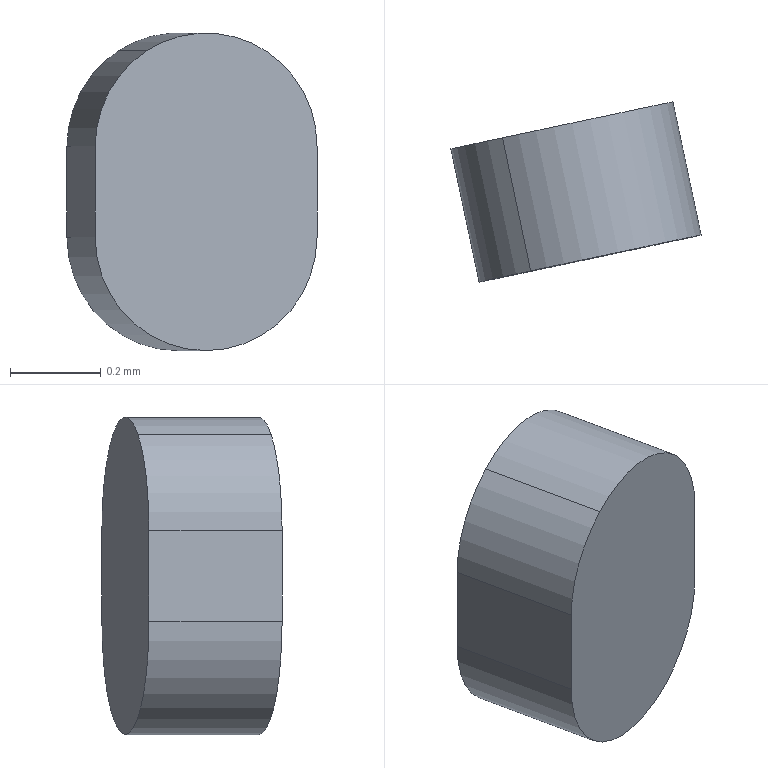Component | SolidWorks | Part31^Assembly1-2 | 1 solid | 7 faces | box 0.55 x 0.4 x 0.7 mm | volume 0 mm3 | plane 4 | cylinder 3 | commonest cylinder face diameters 0.5 x3
STEP:
#1=COLOUR_RGB('',0.7922,0.8196,0.9333);
#2=FILL_AREA_STYLE_COLOUR('',#1);
#3=FILL_AREA_STYLE('',(#2));
#4=SURFACE_STYLE_FILL_AREA(#3);
#5=SURFACE_SIDE_STYLE('',(#4));
#6=SURFACE_STYLE_USAGE(.BOTH.,#5);
#7=PRESENTATION_STYLE_ASSIGNMENT((#6));
#8=CARTESIAN_POINT('',(0.2261,-0.1617,0.1879));
#9=VERTEX_POINT('',#8);
#10=CARTESIAN_POINT('',(0.2408,-0.1586,0.1796));
#11=VERTEX_POINT('',#10);
#12=CARTESIAN_POINT('',(0.2312,-0.1606,0.1796));
#13=DIRECTION('',(-0.2075,0.9782,0.));
#14=DIRECTION('',(0.5246,0.1113,-0.8441));
#15=AXIS2_PLACEMENT_3D('',#12,#13,#14);
#16=CIRCLE('',#15,0.009843);
#17=EDGE_CURVE('',#9,#11,#16,.T.);
#18=ORIENTED_EDGE('',*,*,#17,.F.);
#19=CARTESIAN_POINT('',(0.2285,-0.1733,0.1879));
#20=VERTEX_POINT('',#19);
#21=CARTESIAN_POINT('',(0.2261,-0.1617,0.1879));
#22=DIRECTION('',(0.2075,-0.9782,-0.));
#23=VECTOR('',#22,39.37);
#24=LINE('',#21,#23);
#25=EDGE_CURVE('',#9,#20,#24,.T.);
#26=ORIENTED_EDGE('',*,*,#25,.T.);
#27=CARTESIAN_POINT('',(0.2433,-0.1701,0.1796));
#28=VERTEX_POINT('',#27);
#29=CARTESIAN_POINT('',(0.2337,-0.1722,0.1796));
#30=DIRECTION('',(-0.2075,0.9782,0.));
#31=DIRECTION('',(0.5246,0.1113,-0.8441));
#32=AXIS2_PLACEMENT_3D('',#29,#30,#31);
#33=CIRCLE('',#32,0.009843);
#34=EDGE_CURVE('',#20,#28,#33,.T.);
#35=ORIENTED_EDGE('',*,*,#34,.T.);
#36=CARTESIAN_POINT('',(0.2408,-0.1586,0.1796));
#37=DIRECTION('',(0.2075,-0.9782,-0.));
#38=VECTOR('',#37,39.37);
#39=LINE('',#36,#38);
#40=EDGE_CURVE('',#11,#28,#39,.T.);
#41=ORIENTED_EDGE('',*,*,#40,.F.);
#42=EDGE_LOOP('',(#18,#26,#35,#41));
#43=FACE_OUTER_BOUND('',#42,.T.);
#44=CARTESIAN_POINT('',(0.2312,-0.1606,0.1796));
#45=DIRECTION('',(0.2075,-0.9782,-0.));
#46=DIRECTION('',(-0.5246,-0.1113,0.8441));
#47=AXIS2_PLACEMENT_3D('',#44,#45,#46);
#48=CYLINDRICAL_SURFACE('',#47,0.009843);
#49=ADVANCED_FACE('',(#43),#48,.T.);
#50=ORIENTED_EDGE('',*,*,#25,.F.);
#51=CARTESIAN_POINT('',(0.2216,-0.1627,0.1796));
#52=VERTEX_POINT('',#51);
#53=CARTESIAN_POINT('',(0.2312,-0.1606,0.1796));
#54=DIRECTION('',(-0.2075,0.9782,0.));
#55=DIRECTION('',(0.5246,0.1113,-0.8441));
#56=AXIS2_PLACEMENT_3D('',#53,#54,#55);
#57=CIRCLE('',#56,0.009843);
#58=EDGE_CURVE('',#52,#9,#57,.T.);
#59=ORIENTED_EDGE('',*,*,#58,.F.);
#60=CARTESIAN_POINT('',(0.224,-0.1742,0.1796));
#61=VERTEX_POINT('',#60);
#62=CARTESIAN_POINT('',(0.2216,-0.1627,0.1796));
#63=DIRECTION('',(0.2075,-0.9782,-0.));
#64=VECTOR('',#63,39.37);
#65=LINE('',#62,#64);
#66=EDGE_CURVE('',#52,#61,#65,.T.);
#67=ORIENTED_EDGE('',*,*,#66,.T.);
#68=CARTESIAN_POINT('',(0.2337,-0.1722,0.1796));
#69=DIRECTION('',(-0.2075,0.9782,0.));
#70=DIRECTION('',(0.5246,0.1113,-0.8441));
#71=AXIS2_PLACEMENT_3D('',#68,#69,#70);
#72=CIRCLE('',#71,0.009843);
#73=EDGE_CURVE('',#61,#20,#72,.T.);
#74=ORIENTED_EDGE('',*,*,#73,.T.);
#75=EDGE_LOOP('',(#50,#59,#67,#74));
#76=FACE_OUTER_BOUND('',#75,.T.);
#77=CARTESIAN_POINT('',(0.2312,-0.1606,0.1796));
#78=DIRECTION('',(0.2075,-0.9782,-0.));
#79=DIRECTION('',(-0.5246,-0.1113,0.8441));
#80=AXIS2_PLACEMENT_3D('',#77,#78,#79);
#81=CYLINDRICAL_SURFACE('',#80,0.009843);
#82=ADVANCED_FACE('',(#76),#81,.T.);
#83=CARTESIAN_POINT('',(0.2433,-0.1701,0.1718));
#84=VERTEX_POINT('',#83);
#85=CARTESIAN_POINT('',(0.2433,-0.1701,0.1796));
#86=DIRECTION('',(-0.,-0.,-1.));
#87=VECTOR('',#86,39.37);
#88=LINE('',#85,#87);
#89=EDGE_CURVE('',#28,#84,#88,.T.);
#90=ORIENTED_EDGE('',*,*,#89,.T.);
#91=CARTESIAN_POINT('',(0.2408,-0.1586,0.1718));
#92=VERTEX_POINT('',#91);
#93=CARTESIAN_POINT('',(0.2408,-0.1586,0.1718));
#94=DIRECTION('',(0.2075,-0.9782,-0.));
#95=VECTOR('',#94,39.37);
#96=LINE('',#93,#95);
#97=EDGE_CURVE('',#92,#84,#96,.T.);
#98=ORIENTED_EDGE('',*,*,#97,.F.);
#99=CARTESIAN_POINT('',(0.2408,-0.1586,0.1796));
#100=DIRECTION('',(-0.,-0.,-1.));
#101=VECTOR('',#100,39.37);
#102=LINE('',#99,#101);
#103=EDGE_CURVE('',#11,#92,#102,.T.);
#104=ORIENTED_EDGE('',*,*,#103,.F.);
#105=ORIENTED_EDGE('',*,*,#40,.T.);
#106=EDGE_LOOP('',(#90,#98,#104,#105));
#107=FACE_OUTER_BOUND('',#106,.T.);
#108=CARTESIAN_POINT('',(0.2408,-0.1586,0.1796));
#109=DIRECTION('',(-0.9782,-0.2075,0.));
#110=DIRECTION('',(0.,0.,1.));
#111=AXIS2_PLACEMENT_3D('',#108,#109,#110);
#112=PLANE('',#111);
#113=ADVANCED_FACE('',(#107),#112,.F.);
#114=CARTESIAN_POINT('',(0.224,-0.1742,0.1718));
#115=VERTEX_POINT('',#114);
#116=CARTESIAN_POINT('',(0.2337,-0.1722,0.1718));
#117=DIRECTION('',(-0.2075,0.9782,0.));
#118=DIRECTION('',(0.5246,0.1113,-0.8441));
#119=AXIS2_PLACEMENT_3D('',#116,#117,#118);
#120=CIRCLE('',#119,0.009843);
#121=EDGE_CURVE('',#84,#115,#120,.T.);
#122=ORIENTED_EDGE('',*,*,#121,.T.);
#123=CARTESIAN_POINT('',(0.2216,-0.1627,0.1718));
#124=VERTEX_POINT('',#123);
#125=CARTESIAN_POINT('',(0.2216,-0.1627,0.1718));
#126=DIRECTION('',(0.2075,-0.9782,-0.));
#127=VECTOR('',#126,39.37);
#128=LINE('',#125,#127);
#129=EDGE_CURVE('',#124,#115,#128,.T.);
#130=ORIENTED_EDGE('',*,*,#129,.F.);
#131=CARTESIAN_POINT('',(0.2312,-0.1606,0.1718));
#132=DIRECTION('',(-0.2075,0.9782,0.));
#133=DIRECTION('',(0.5246,0.1113,-0.8441));
#134=AXIS2_PLACEMENT_3D('',#131,#132,#133);
#135=CIRCLE('',#134,0.009843);
#136=EDGE_CURVE('',#92,#124,#135,.T.);
#137=ORIENTED_EDGE('',*,*,#136,.F.);
#138=ORIENTED_EDGE('',*,*,#97,.T.);
#139=EDGE_LOOP('',(#122,#130,#137,#138));
#140=FACE_OUTER_BOUND('',#139,.T.);
#141=CARTESIAN_POINT('',(0.2312,-0.1606,0.1718));
#142=DIRECTION('',(0.2075,-0.9782,-0.));
#143=DIRECTION('',(-0.5246,-0.1113,0.8441));
#144=AXIS2_PLACEMENT_3D('',#141,#142,#143);
#145=CYLINDRICAL_SURFACE('',#144,0.009843);
#146=ADVANCED_FACE('',(#140),#145,.T.);
#147=CARTESIAN_POINT('',(0.224,-0.1742,0.1796));
#148=DIRECTION('',(0.,0.,1.));
#149=VECTOR('',#148,39.37);
#150=LINE('',#147,#149);
#151=EDGE_CURVE('',#115,#61,#150,.T.);
#152=ORIENTED_EDGE('',*,*,#151,.T.);
#153=ORIENTED_EDGE('',*,*,#66,.F.);
#154=CARTESIAN_POINT('',(0.2216,-0.1627,0.1796));
#155=DIRECTION('',(0.,0.,1.));
#156=VECTOR('',#155,39.37);
#157=LINE('',#154,#156);
#158=EDGE_CURVE('',#124,#52,#157,.T.);
#159=ORIENTED_EDGE('',*,*,#158,.F.);
#160=ORIENTED_EDGE('',*,*,#129,.T.);
#161=EDGE_LOOP('',(#152,#153,#159,#160));
#162=FACE_OUTER_BOUND('',#161,.T.);
#163=CARTESIAN_POINT('',(0.2216,-0.1627,0.1796));
#164=DIRECTION('',(0.9782,0.2075,-0.));
#165=DIRECTION('',(-0.,-0.,-1.));
#166=AXIS2_PLACEMENT_3D('',#163,#164,#165);
#167=PLANE('',#166);
#168=ADVANCED_FACE('',(#162),#167,.F.);
#169=ORIENTED_EDGE('',*,*,#58,.T.);
#170=ORIENTED_EDGE('',*,*,#17,.T.);
#171=ORIENTED_EDGE('',*,*,#103,.T.);
#172=ORIENTED_EDGE('',*,*,#136,.T.);
#173=ORIENTED_EDGE('',*,*,#158,.T.);
#174=EDGE_LOOP('',(#169,#170,#171,#172,#173));
#175=FACE_OUTER_BOUND('',#174,.T.);
#176=CARTESIAN_POINT('',(0.2312,-0.1606,0.1796));
#177=DIRECTION('',(-0.2075,0.9782,0.));
#178=DIRECTION('',(0.5246,0.1113,-0.8441));
#179=AXIS2_PLACEMENT_3D('',#176,#177,#178);
#180=PLANE('',#179);
#181=ADVANCED_FACE('',(#175),#180,.T.);
#182=ORIENTED_EDGE('',*,*,#73,.F.);
#183=ORIENTED_EDGE('',*,*,#151,.F.);
#184=ORIENTED_EDGE('',*,*,#121,.F.);
#185=ORIENTED_EDGE('',*,*,#89,.F.);
#186=ORIENTED_EDGE('',*,*,#34,.F.);
#187=EDGE_LOOP('',(#182,#183,#184,#185,#186));
#188=FACE_OUTER_BOUND('',#187,.T.);
#189=CARTESIAN_POINT('',(0.2337,-0.1722,0.1796));
#190=DIRECTION('',(-0.2075,0.9782,0.));
#191=DIRECTION('',(0.5246,0.1113,-0.8441));
#192=AXIS2_PLACEMENT_3D('',#189,#190,#191);
#193=PLANE('',#192);
#194=ADVANCED_FACE('',(#188),#193,.F.);
#195=CLOSED_SHELL('',(#49,#82,#113,#146,#168,#181,#194));
#196=MANIFOLD_SOLID_BREP('',#195);
#197=STYLED_ITEM('',(#7),#196);
#198=PRESENTATION_LAYER_ASSIGNMENT('','',(#197));
#199=CARTESIAN_POINT('',(0.,0.,0.));
#200=DIRECTION('',(0.,0.,1.));
#201=DIRECTION('',(1.,0.,0.));
#202=AXIS2_PLACEMENT_3D('',#199,#200,#201);
#203=(LENGTH_UNIT()NAMED_UNIT(*)SI_UNIT($,.METRE.));
#204=LENGTH_MEASURE_WITH_UNIT(LENGTH_MEASURE(0.0254),#203);
#205=DIMENSIONAL_EXPONENTS(1.,0.,0.,0.,0.,0.,0.);
#206=(CONVERSION_BASED_UNIT('',#204)LENGTH_UNIT()NAMED_UNIT(#205));
#207=UNCERTAINTY_MEASURE_WITH_UNIT(LENGTH_MEASURE(0.00001),#206,'','');
#208=(NAMED_UNIT(*)PLANE_ANGLE_UNIT()SI_UNIT($,.RADIAN.));
#209=(NAMED_UNIT(*)SI_UNIT($,.STERADIAN.)SOLID_ANGLE_UNIT());
#210=(GEOMETRIC_REPRESENTATION_CONTEXT(3)GLOBAL_UNCERTAINTY_ASSIGNED_CONTEXT((#207))GLOBAL_UNIT_ASSIGNED_CONTEXT((#206,#208,#209))REPRESENTATION_CONTEXT('',''));
#211=ADVANCED_BREP_SHAPE_REPRESENTATION('',(#196,#202),#210);
#212=(LENGTH_UNIT()NAMED_UNIT(*)SI_UNIT($,.METRE.));
#213=LENGTH_MEASURE_WITH_UNIT(LENGTH_MEASURE(0.0254),#212);
#214=DIMENSIONAL_EXPONENTS(1.,0.,0.,0.,0.,0.,0.);
#215=(CONVERSION_BASED_UNIT('',#213)LENGTH_UNIT()NAMED_UNIT(#214));
#216=UNCERTAINTY_MEASURE_WITH_UNIT(LENGTH_MEASURE(0.00001),#215,'','');
#217=(NAMED_UNIT(*)PLANE_ANGLE_UNIT()SI_UNIT($,.RADIAN.));
#218=(NAMED_UNIT(*)SI_UNIT($,.STERADIAN.)SOLID_ANGLE_UNIT());
#219=(GEOMETRIC_REPRESENTATION_CONTEXT(3)GLOBAL_UNCERTAINTY_ASSIGNED_CONTEXT((#216))GLOBAL_UNIT_ASSIGNED_CONTEXT((#215,#217,#218))REPRESENTATION_CONTEXT('',''));
#220=MECHANICAL_DESIGN_GEOMETRIC_PRESENTATION_REPRESENTATION('',(#197),#219);